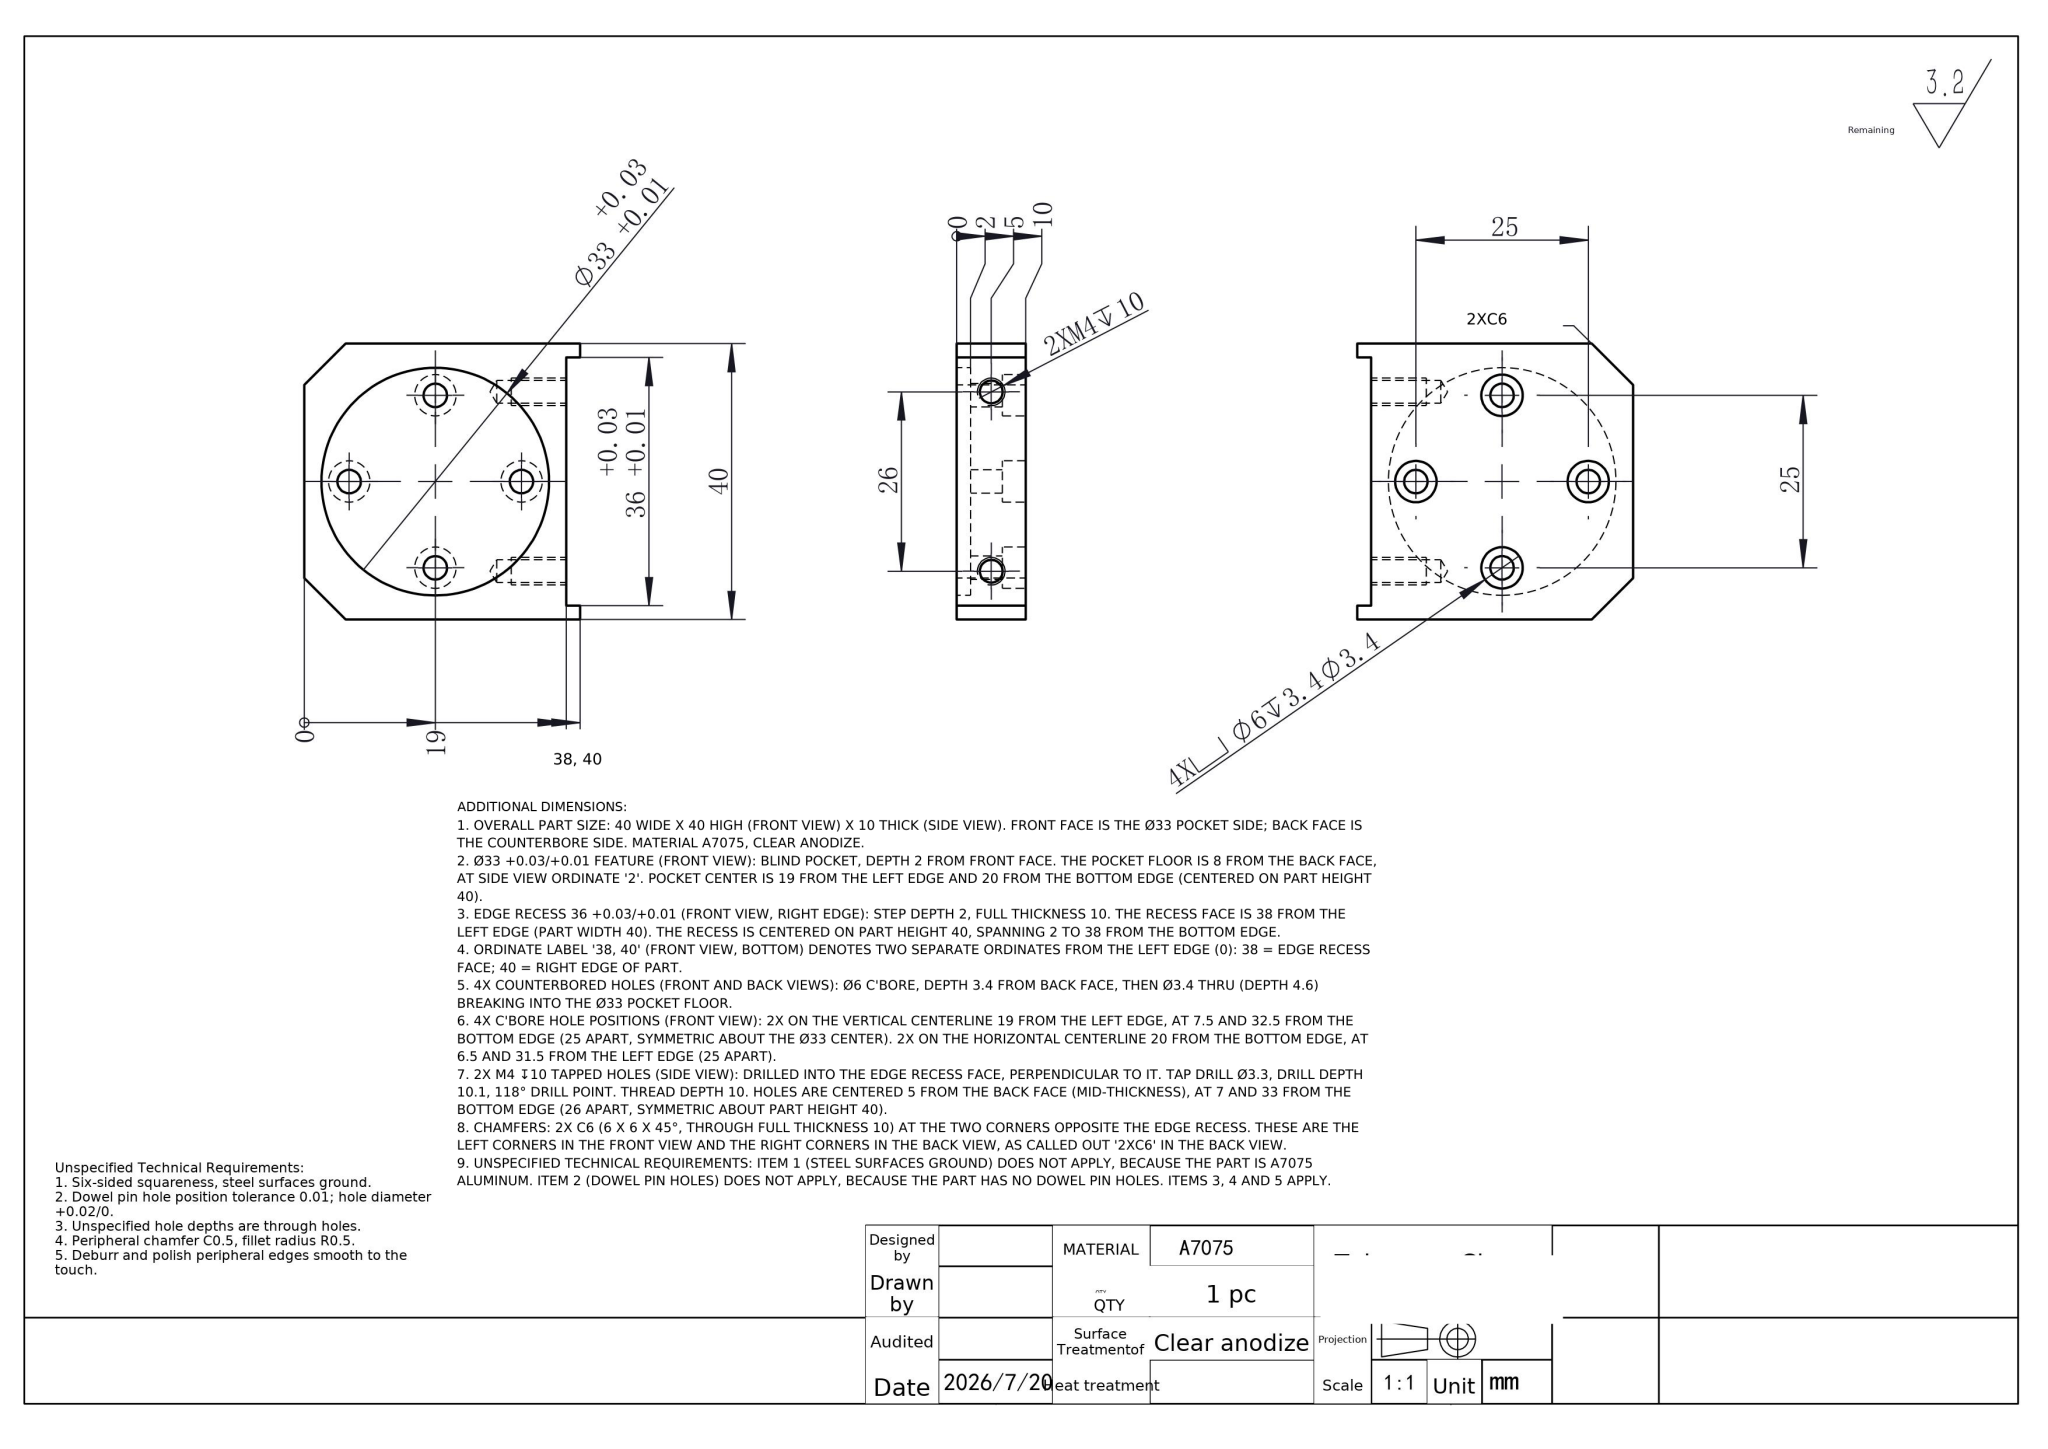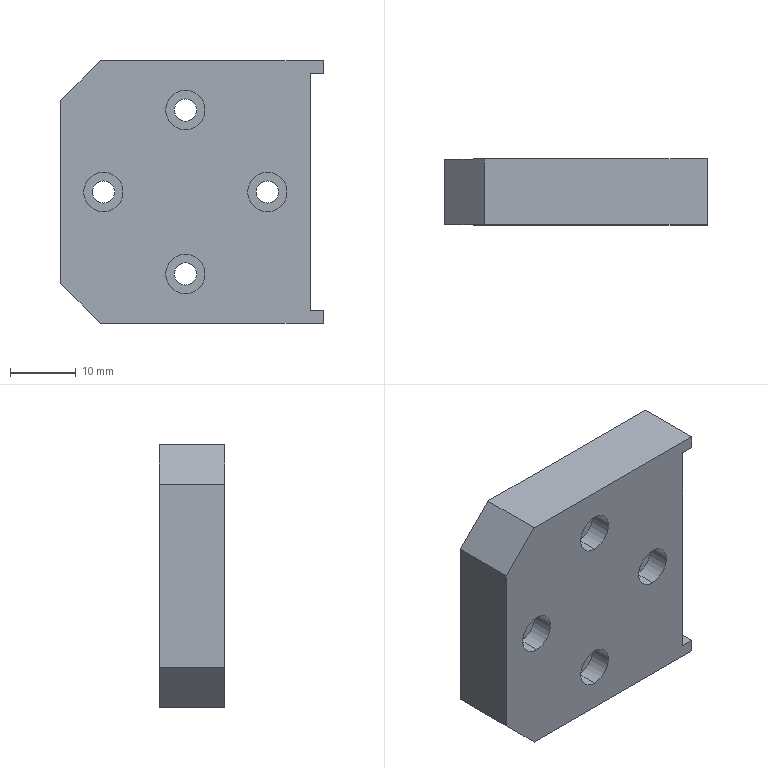Part | NX | mm | 1 solid | 43 faces | box 40 x 10 x 40 mm | volume 12479 mm3 | cylinder 22 | plane 17 | cone 4 | commonest cylinder face diameters 6 x8 3.4 x8 3.3 x4 33 x2